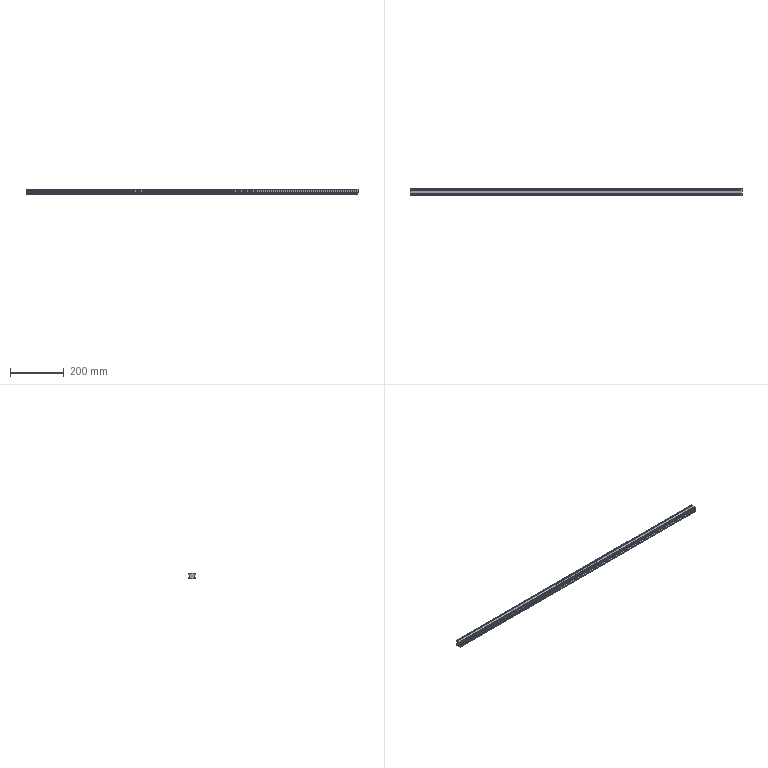Component | SolidWorks | GuideRailHGH25-1 | 1 solid | 34 faces | box 1240 x 23 x 22 mm | volume 545518 mm3 | plane 30 | cylinder 4 | commonest cylinder face diameters 4.6 x4
build123d program:
from build123d import *

# Parameters (mm, degrees)
BOSS_EXTRUDE1_DEPTH = 620


with BuildPart() as part:
    # Sketch1 → Boss-Extrude1 (new, symmetric)
    with BuildSketch(Plane.XY):
        with BuildLine():
            Line((-10.5, 0), (-8.214, 0))
            Line((-8.214, 0), (-7.448, 0.7667))
            Line((-7.448, 0.7667), (-5.695, 0.7667))
            Line((-5.695, 0.7667), (-4.929, 0))
            Line((-4.929, 0), (4.929, 0))
            Line((4.929, 0), (5.695, 0.7667))
            Line((5.695, 0.7667), (7.448, 0.7667))
            Line((7.448, 0.7667), (8.214, 0))
            Line((8.214, 0), (10.5, 0))
            Line((10.5, 0), (11.5, 1))
            Line((11.5, 1), (11.5, 5.5))
            Line((11.5, 5.5), (8.05, 8.95))
            Line((8.05, 8.95), (8.05, 11.95))
            Line((8.05, 11.95), (8.699, 12.599))
            ThreePointArc((8.699, 12.599), (9.368, 14.082), (10.851, 14.751))
            Line((10.851, 14.751), (11.5, 15.4))
            Line((11.5, 15.4), (11.5, 18.55))
            Line((11.5, 18.55), (10.851, 19.199))
            ThreePointArc((10.851, 19.199), (9.368, 19.868), (8.699, 21.351))
            Line((8.699, 21.351), (8.05, 22))
            Line((8.05, 22), (-8.05, 22))
            Line((-8.05, 22), (-8.699, 21.351))
            ThreePointArc((-8.699, 21.351), (-9.368, 19.868), (-10.851, 19.199))
            Line((-10.851, 19.199), (-11.5, 18.55))
            Line((-11.5, 18.55), (-11.5, 15.4))
            Line((-11.5, 15.4), (-10.851, 14.751))
            ThreePointArc((-10.851, 14.751), (-9.368, 14.082), (-8.699, 12.599))
            Line((-8.699, 12.599), (-8.05, 11.95))
            Line((-8.05, 11.95), (-8.05, 8.95))
            Line((-8.05, 8.95), (-11.5, 5.5))
            Line((-11.5, 5.5), (-11.5, 1))
            Line((-11.5, 1), (-10.5, 0))
        make_face()
    extrude(amount=BOSS_EXTRUDE1_DEPTH, both=True)


solid = part.part

# Placed as in the assembly
solid = solid.moved(Location((160, -213.5, 69), (-90, 90, 0)))
STEP:
#1=CARTESIAN_POINT('',(-18.11,-8.748,1.876));
#2=VERTEX_POINT('',#1);
#3=CARTESIAN_POINT('',(-18.11,-8.722,1.85));
#4=VERTEX_POINT('',#3);
#5=CARTESIAN_POINT('',(-18.11,-8.748,1.876));
#6=DIRECTION('',(-0.,0.7071,-0.7071));
#7=VECTOR('',#6,39.37);
#8=LINE('',#5,#7);
#9=EDGE_CURVE('',#2,#4,#8,.T.);
#10=ORIENTED_EDGE('',*,*,#9,.T.);
#11=CARTESIAN_POINT('',(30.709,-8.722,1.85));
#12=VERTEX_POINT('',#11);
#13=CARTESIAN_POINT('',(30.709,-8.722,1.85));
#14=DIRECTION('',(-1.,0.,0.));
#15=VECTOR('',#14,39.37);
#16=LINE('',#13,#15);
#17=EDGE_CURVE('',#12,#4,#16,.T.);
#18=ORIENTED_EDGE('',*,*,#17,.F.);
#19=CARTESIAN_POINT('',(30.709,-8.748,1.876));
#20=VERTEX_POINT('',#19);
#21=CARTESIAN_POINT('',(30.709,-8.748,1.876));
#22=DIRECTION('',(-0.,0.7071,-0.7071));
#23=VECTOR('',#22,39.37);
#24=LINE('',#21,#23);
#25=EDGE_CURVE('',#20,#12,#24,.T.);
#26=ORIENTED_EDGE('',*,*,#25,.F.);
#27=CARTESIAN_POINT('',(30.709,-8.748,1.876));
#28=DIRECTION('',(-1.,0.,0.));
#29=VECTOR('',#28,39.37);
#30=LINE('',#27,#29);
#31=EDGE_CURVE('',#20,#2,#30,.T.);
#32=ORIENTED_EDGE('',*,*,#31,.T.);
#33=EDGE_LOOP('',(#10,#18,#26,#32));
#34=FACE_OUTER_BOUND('',#33,.T.);
#35=CARTESIAN_POINT('',(30.709,-8.748,1.876));
#36=DIRECTION('',(0.,0.7071,0.7071));
#37=DIRECTION('',(0.,-0.7071,0.7071));
#38=AXIS2_PLACEMENT_3D('',#35,#36,#37);
#39=PLANE('',#38);
#40=ADVANCED_FACE('',(#34),#39,.F.);
#41=CARTESIAN_POINT('',(-18.11,-8.089,1.85));
#42=VERTEX_POINT('',#41);
#43=CARTESIAN_POINT('',(-18.11,-8.722,1.85));
#44=DIRECTION('',(0.,1.,0.));
#45=VECTOR('',#44,39.37);
#46=LINE('',#43,#45);
#47=EDGE_CURVE('',#4,#42,#46,.T.);
#48=ORIENTED_EDGE('',*,*,#47,.T.);
#49=CARTESIAN_POINT('',(30.709,-8.089,1.85));
#50=VERTEX_POINT('',#49);
#51=CARTESIAN_POINT('',(30.709,-8.089,1.85));
#52=DIRECTION('',(-1.,0.,0.));
#53=VECTOR('',#52,39.37);
#54=LINE('',#51,#53);
#55=EDGE_CURVE('',#50,#42,#54,.T.);
#56=ORIENTED_EDGE('',*,*,#55,.F.);
#57=CARTESIAN_POINT('',(30.709,-8.722,1.85));
#58=DIRECTION('',(0.,1.,0.));
#59=VECTOR('',#58,39.37);
#60=LINE('',#57,#59);
#61=EDGE_CURVE('',#12,#50,#60,.T.);
#62=ORIENTED_EDGE('',*,*,#61,.F.);
#63=ORIENTED_EDGE('',*,*,#17,.T.);
#64=EDGE_LOOP('',(#48,#56,#62,#63));
#65=FACE_OUTER_BOUND('',#64,.T.);
#66=CARTESIAN_POINT('',(30.709,-8.722,1.85));
#67=DIRECTION('',(0.,-0.,1.));
#68=DIRECTION('',(-0.,-1.,-0.));
#69=AXIS2_PLACEMENT_3D('',#66,#67,#68);
#70=PLANE('',#69);
#71=ADVANCED_FACE('',(#65),#70,.F.);
#72=CARTESIAN_POINT('',(-18.11,-8.063,1.876));
#73=VERTEX_POINT('',#72);
#74=CARTESIAN_POINT('',(-18.11,-8.089,1.85));
#75=DIRECTION('',(0.,0.7071,0.7071));
#76=VECTOR('',#75,39.37);
#77=LINE('',#74,#76);
#78=EDGE_CURVE('',#42,#73,#77,.T.);
#79=ORIENTED_EDGE('',*,*,#78,.T.);
#80=CARTESIAN_POINT('',(30.709,-8.063,1.876));
#81=VERTEX_POINT('',#80);
#82=CARTESIAN_POINT('',(30.709,-8.063,1.876));
#83=DIRECTION('',(-1.,0.,0.));
#84=VECTOR('',#83,39.37);
#85=LINE('',#82,#84);
#86=EDGE_CURVE('',#81,#73,#85,.T.);
#87=ORIENTED_EDGE('',*,*,#86,.F.);
#88=CARTESIAN_POINT('',(30.709,-8.089,1.85));
#89=DIRECTION('',(0.,0.7071,0.7071));
#90=VECTOR('',#89,39.37);
#91=LINE('',#88,#90);
#92=EDGE_CURVE('',#50,#81,#91,.T.);
#93=ORIENTED_EDGE('',*,*,#92,.F.);
#94=ORIENTED_EDGE('',*,*,#55,.T.);
#95=EDGE_LOOP('',(#79,#87,#93,#94));
#96=FACE_OUTER_BOUND('',#95,.T.);
#97=CARTESIAN_POINT('',(30.709,-8.089,1.85));
#98=DIRECTION('',(0.,-0.7071,0.7071));
#99=DIRECTION('',(-0.,-0.7071,-0.7071));
#100=AXIS2_PLACEMENT_3D('',#97,#98,#99);
#101=PLANE('',#100);
#102=ADVANCED_FACE('',(#96),#101,.F.);
#103=CARTESIAN_POINT('',(-18.11,-7.978,1.961));
#104=VERTEX_POINT('',#103);
#105=CARTESIAN_POINT('',(-18.11,-7.973,1.87));
#106=DIRECTION('',(1.,-0.,-0.));
#107=DIRECTION('',(0.,-1.,-0.));
#108=AXIS2_PLACEMENT_3D('',#105,#106,#107);
#109=CIRCLE('',#108,0.09055);
#110=EDGE_CURVE('',#104,#73,#109,.T.);
#111=ORIENTED_EDGE('',*,*,#110,.F.);
#112=CARTESIAN_POINT('',(30.709,-7.978,1.961));
#113=VERTEX_POINT('',#112);
#114=CARTESIAN_POINT('',(30.709,-7.978,1.961));
#115=DIRECTION('',(-1.,0.,0.));
#116=VECTOR('',#115,39.37);
#117=LINE('',#114,#116);
#118=EDGE_CURVE('',#113,#104,#117,.T.);
#119=ORIENTED_EDGE('',*,*,#118,.F.);
#120=CARTESIAN_POINT('',(30.709,-7.973,1.87));
#121=DIRECTION('',(1.,-0.,-0.));
#122=DIRECTION('',(0.,-1.,-0.));
#123=AXIS2_PLACEMENT_3D('',#120,#121,#122);
#124=CIRCLE('',#123,0.09055);
#125=EDGE_CURVE('',#113,#81,#124,.T.);
#126=ORIENTED_EDGE('',*,*,#125,.T.);
#127=ORIENTED_EDGE('',*,*,#86,.T.);
#128=EDGE_LOOP('',(#111,#119,#126,#127));
#129=FACE_OUTER_BOUND('',#128,.T.);
#130=CARTESIAN_POINT('',(30.709,-7.973,1.87));
#131=DIRECTION('',(-1.,0.,0.));
#132=DIRECTION('',(0.,1.,0.));
#133=AXIS2_PLACEMENT_3D('',#130,#131,#132);
#134=CYLINDRICAL_SURFACE('',#133,0.09055);
#135=ADVANCED_FACE('',(#129),#134,.F.);
#136=CARTESIAN_POINT('',(-18.11,-7.953,1.986));
#137=VERTEX_POINT('',#136);
#138=CARTESIAN_POINT('',(-18.11,-7.978,1.961));
#139=DIRECTION('',(0.,0.7071,0.7071));
#140=VECTOR('',#139,39.37);
#141=LINE('',#138,#140);
#142=EDGE_CURVE('',#104,#137,#141,.T.);
#143=ORIENTED_EDGE('',*,*,#142,.T.);
#144=CARTESIAN_POINT('',(30.709,-7.953,1.986));
#145=VERTEX_POINT('',#144);
#146=CARTESIAN_POINT('',(30.709,-7.953,1.986));
#147=DIRECTION('',(-1.,0.,0.));
#148=VECTOR('',#147,39.37);
#149=LINE('',#146,#148);
#150=EDGE_CURVE('',#145,#137,#149,.T.);
#151=ORIENTED_EDGE('',*,*,#150,.F.);
#152=CARTESIAN_POINT('',(30.709,-7.978,1.961));
#153=DIRECTION('',(0.,0.7071,0.7071));
#154=VECTOR('',#153,39.37);
#155=LINE('',#152,#154);
#156=EDGE_CURVE('',#113,#145,#155,.T.);
#157=ORIENTED_EDGE('',*,*,#156,.F.);
#158=ORIENTED_EDGE('',*,*,#118,.T.);
#159=EDGE_LOOP('',(#143,#151,#157,#158));
#160=FACE_OUTER_BOUND('',#159,.T.);
#161=CARTESIAN_POINT('',(30.709,-7.978,1.961));
#162=DIRECTION('',(0.,-0.7071,0.7071));
#163=DIRECTION('',(-0.,-0.7071,-0.7071));
#164=AXIS2_PLACEMENT_3D('',#161,#162,#163);
#165=PLANE('',#164);
#166=ADVANCED_FACE('',(#160),#165,.F.);
#167=CARTESIAN_POINT('',(-18.11,-7.953,2.11));
#168=VERTEX_POINT('',#167);
#169=CARTESIAN_POINT('',(-18.11,-7.953,1.986));
#170=DIRECTION('',(0.,-0.,1.));
#171=VECTOR('',#170,39.37);
#172=LINE('',#169,#171);
#173=EDGE_CURVE('',#137,#168,#172,.T.);
#174=ORIENTED_EDGE('',*,*,#173,.T.);
#175=CARTESIAN_POINT('',(30.709,-7.953,2.11));
#176=VERTEX_POINT('',#175);
#177=CARTESIAN_POINT('',(30.709,-7.953,2.11));
#178=DIRECTION('',(-1.,0.,0.));
#179=VECTOR('',#178,39.37);
#180=LINE('',#177,#179);
#181=EDGE_CURVE('',#176,#168,#180,.T.);
#182=ORIENTED_EDGE('',*,*,#181,.F.);
#183=CARTESIAN_POINT('',(30.709,-7.953,1.986));
#184=DIRECTION('',(0.,-0.,1.));
#185=VECTOR('',#184,39.37);
#186=LINE('',#183,#185);
#187=EDGE_CURVE('',#145,#176,#186,.T.);
#188=ORIENTED_EDGE('',*,*,#187,.F.);
#189=ORIENTED_EDGE('',*,*,#150,.T.);
#190=EDGE_LOOP('',(#174,#182,#188,#189));
#191=FACE_OUTER_BOUND('',#190,.T.);
#192=CARTESIAN_POINT('',(30.709,-7.953,1.986));
#193=DIRECTION('',(-0.,-1.,-0.));
#194=DIRECTION('',(-1.,0.,0.));
#195=AXIS2_PLACEMENT_3D('',#192,#193,#194);
#196=PLANE('',#195);
#197=ADVANCED_FACE('',(#191),#196,.F.);
#198=CARTESIAN_POINT('',(-18.11,-7.978,2.136));
#199=VERTEX_POINT('',#198);
#200=CARTESIAN_POINT('',(-18.11,-7.953,2.11));
#201=DIRECTION('',(0.,-0.7071,0.7071));
#202=VECTOR('',#201,39.37);
#203=LINE('',#200,#202);
#204=EDGE_CURVE('',#168,#199,#203,.T.);
#205=ORIENTED_EDGE('',*,*,#204,.T.);
#206=CARTESIAN_POINT('',(30.709,-7.978,2.136));
#207=VERTEX_POINT('',#206);
#208=CARTESIAN_POINT('',(30.709,-7.978,2.136));
#209=DIRECTION('',(-1.,0.,0.));
#210=VECTOR('',#209,39.37);
#211=LINE('',#208,#210);
#212=EDGE_CURVE('',#207,#199,#211,.T.);
#213=ORIENTED_EDGE('',*,*,#212,.F.);
#214=CARTESIAN_POINT('',(30.709,-7.953,2.11));
#215=DIRECTION('',(0.,-0.7071,0.7071));
#216=VECTOR('',#215,39.37);
#217=LINE('',#214,#216);
#218=EDGE_CURVE('',#176,#207,#217,.T.);
#219=ORIENTED_EDGE('',*,*,#218,.F.);
#220=ORIENTED_EDGE('',*,*,#181,.T.);
#221=EDGE_LOOP('',(#205,#213,#219,#220));
#222=FACE_OUTER_BOUND('',#221,.T.);
#223=CARTESIAN_POINT('',(30.709,-7.953,2.11));
#224=DIRECTION('',(-0.,-0.7071,-0.7071));
#225=DIRECTION('',(-0.,0.7071,-0.7071));
#226=AXIS2_PLACEMENT_3D('',#223,#224,#225);
#227=PLANE('',#226);
#228=ADVANCED_FACE('',(#222),#227,.F.);
#229=CARTESIAN_POINT('',(-18.11,-8.063,2.221));
#230=VERTEX_POINT('',#229);
#231=CARTESIAN_POINT('',(-18.11,-7.973,2.226));
#232=DIRECTION('',(1.,-0.,-0.));
#233=DIRECTION('',(0.,-1.,-0.));
#234=AXIS2_PLACEMENT_3D('',#231,#232,#233);
#235=CIRCLE('',#234,0.09055);
#236=EDGE_CURVE('',#230,#199,#235,.T.);
#237=ORIENTED_EDGE('',*,*,#236,.F.);
#238=CARTESIAN_POINT('',(30.709,-8.063,2.221));
#239=VERTEX_POINT('',#238);
#240=CARTESIAN_POINT('',(30.709,-8.063,2.221));
#241=DIRECTION('',(-1.,0.,0.));
#242=VECTOR('',#241,39.37);
#243=LINE('',#240,#242);
#244=EDGE_CURVE('',#239,#230,#243,.T.);
#245=ORIENTED_EDGE('',*,*,#244,.F.);
#246=CARTESIAN_POINT('',(30.709,-7.973,2.226));
#247=DIRECTION('',(1.,-0.,-0.));
#248=DIRECTION('',(0.,-1.,-0.));
#249=AXIS2_PLACEMENT_3D('',#246,#247,#248);
#250=CIRCLE('',#249,0.09055);
#251=EDGE_CURVE('',#239,#207,#250,.T.);
#252=ORIENTED_EDGE('',*,*,#251,.T.);
#253=ORIENTED_EDGE('',*,*,#212,.T.);
#254=EDGE_LOOP('',(#237,#245,#252,#253));
#255=FACE_OUTER_BOUND('',#254,.T.);
#256=CARTESIAN_POINT('',(30.709,-7.973,2.226));
#257=DIRECTION('',(-1.,0.,0.));
#258=DIRECTION('',(0.,1.,0.));
#259=AXIS2_PLACEMENT_3D('',#256,#257,#258);
#260=CYLINDRICAL_SURFACE('',#259,0.09055);
#261=ADVANCED_FACE('',(#255),#260,.F.);
#262=CARTESIAN_POINT('',(-18.11,-8.089,2.246));
#263=VERTEX_POINT('',#262);
#264=CARTESIAN_POINT('',(-18.11,-8.063,2.221));
#265=DIRECTION('',(0.,-0.7071,0.7071));
#266=VECTOR('',#265,39.37);
#267=LINE('',#264,#266);
#268=EDGE_CURVE('',#230,#263,#267,.T.);
#269=ORIENTED_EDGE('',*,*,#268,.T.);
#270=CARTESIAN_POINT('',(30.709,-8.089,2.246));
#271=VERTEX_POINT('',#270);
#272=CARTESIAN_POINT('',(30.709,-8.089,2.246));
#273=DIRECTION('',(-1.,0.,0.));
#274=VECTOR('',#273,39.37);
#275=LINE('',#272,#274);
#276=EDGE_CURVE('',#271,#263,#275,.T.);
#277=ORIENTED_EDGE('',*,*,#276,.F.);
#278=CARTESIAN_POINT('',(30.709,-8.063,2.221));
#279=DIRECTION('',(0.,-0.7071,0.7071));
#280=VECTOR('',#279,39.37);
#281=LINE('',#278,#280);
#282=EDGE_CURVE('',#239,#271,#281,.T.);
#283=ORIENTED_EDGE('',*,*,#282,.F.);
#284=ORIENTED_EDGE('',*,*,#244,.T.);
#285=EDGE_LOOP('',(#269,#277,#283,#284));
#286=FACE_OUTER_BOUND('',#285,.T.);
#287=CARTESIAN_POINT('',(30.709,-8.063,2.221));
#288=DIRECTION('',(-0.,-0.7071,-0.7071));
#289=DIRECTION('',(-0.,0.7071,-0.7071));
#290=AXIS2_PLACEMENT_3D('',#287,#288,#289);
#291=PLANE('',#290);
#292=ADVANCED_FACE('',(#286),#291,.F.);
#293=CARTESIAN_POINT('',(-18.11,-8.089,2.364));
#294=VERTEX_POINT('',#293);
#295=CARTESIAN_POINT('',(-18.11,-8.089,2.246));
#296=DIRECTION('',(0.,-0.,1.));
#297=VECTOR('',#296,39.37);
#298=LINE('',#295,#297);
#299=EDGE_CURVE('',#263,#294,#298,.T.);
#300=ORIENTED_EDGE('',*,*,#299,.T.);
#301=CARTESIAN_POINT('',(30.709,-8.089,2.364));
#302=VERTEX_POINT('',#301);
#303=CARTESIAN_POINT('',(30.709,-8.089,2.364));
#304=DIRECTION('',(-1.,0.,0.));
#305=VECTOR('',#304,39.37);
#306=LINE('',#303,#305);
#307=EDGE_CURVE('',#302,#294,#306,.T.);
#308=ORIENTED_EDGE('',*,*,#307,.F.);
#309=CARTESIAN_POINT('',(30.709,-8.089,2.246));
#310=DIRECTION('',(0.,-0.,1.));
#311=VECTOR('',#310,39.37);
#312=LINE('',#309,#311);
#313=EDGE_CURVE('',#271,#302,#312,.T.);
#314=ORIENTED_EDGE('',*,*,#313,.F.);
#315=ORIENTED_EDGE('',*,*,#276,.T.);
#316=EDGE_LOOP('',(#300,#308,#314,#315));
#317=FACE_OUTER_BOUND('',#316,.T.);
#318=CARTESIAN_POINT('',(30.709,-8.089,2.246));
#319=DIRECTION('',(-0.,-1.,-0.));
#320=DIRECTION('',(-0.,0.,-1.));
#321=AXIS2_PLACEMENT_3D('',#318,#319,#320);
#322=PLANE('',#321);
#323=ADVANCED_FACE('',(#317),#322,.F.);
#324=CARTESIAN_POINT('',(-18.11,-7.953,2.5));
#325=VERTEX_POINT('',#324);
#326=CARTESIAN_POINT('',(-18.11,-8.089,2.364));
#327=DIRECTION('',(0.,0.7071,0.7071));
#328=VECTOR('',#327,39.37);
#329=LINE('',#326,#328);
#330=EDGE_CURVE('',#294,#325,#329,.T.);
#331=ORIENTED_EDGE('',*,*,#330,.T.);
#332=CARTESIAN_POINT('',(30.709,-7.953,2.5));
#333=VERTEX_POINT('',#332);
#334=CARTESIAN_POINT('',(30.709,-7.953,2.5));
#335=DIRECTION('',(-1.,0.,0.));
#336=VECTOR('',#335,39.37);
#337=LINE('',#334,#336);
#338=EDGE_CURVE('',#333,#325,#337,.T.);
#339=ORIENTED_EDGE('',*,*,#338,.F.);
#340=CARTESIAN_POINT('',(30.709,-8.089,2.364));
#341=DIRECTION('',(0.,0.7071,0.7071));
#342=VECTOR('',#341,39.37);
#343=LINE('',#340,#342);
#344=EDGE_CURVE('',#302,#333,#343,.T.);
#345=ORIENTED_EDGE('',*,*,#344,.F.);
#346=ORIENTED_EDGE('',*,*,#307,.T.);
#347=EDGE_LOOP('',(#331,#339,#345,#346));
#348=FACE_OUTER_BOUND('',#347,.T.);
#349=CARTESIAN_POINT('',(30.709,-8.089,2.364));
#350=DIRECTION('',(0.,-0.7071,0.7071));
#351=DIRECTION('',(-0.,-0.7071,-0.7071));
#352=AXIS2_PLACEMENT_3D('',#349,#350,#351);
#353=PLANE('',#352);
#354=ADVANCED_FACE('',(#348),#353,.F.);
#355=CARTESIAN_POINT('',(-18.11,-7.953,2.677));
#356=VERTEX_POINT('',#355);
#357=CARTESIAN_POINT('',(-18.11,-7.953,2.5));
#358=DIRECTION('',(0.,-0.,1.));
#359=VECTOR('',#358,39.37);
#360=LINE('',#357,#359);
#361=EDGE_CURVE('',#325,#356,#360,.T.);
#362=ORIENTED_EDGE('',*,*,#361,.T.);
#363=CARTESIAN_POINT('',(30.709,-7.953,2.677));
#364=VERTEX_POINT('',#363);
#365=CARTESIAN_POINT('',(30.709,-7.953,2.677));
#366=DIRECTION('',(-1.,0.,0.));
#367=VECTOR('',#366,39.37);
#368=LINE('',#365,#367);
#369=EDGE_CURVE('',#364,#356,#368,.T.);
#370=ORIENTED_EDGE('',*,*,#369,.F.);
#371=CARTESIAN_POINT('',(30.709,-7.953,2.5));
#372=DIRECTION('',(0.,-0.,1.));
#373=VECTOR('',#372,39.37);
#374=LINE('',#371,#373);
#375=EDGE_CURVE('',#333,#364,#374,.T.);
#376=ORIENTED_EDGE('',*,*,#375,.F.);
#377=ORIENTED_EDGE('',*,*,#338,.T.);
#378=EDGE_LOOP('',(#362,#370,#376,#377));
#379=FACE_OUTER_BOUND('',#378,.T.);
#380=CARTESIAN_POINT('',(30.709,-7.953,2.5));
#381=DIRECTION('',(-0.,-1.,-0.));
#382=DIRECTION('',(-1.,0.,0.));
#383=AXIS2_PLACEMENT_3D('',#380,#381,#382);
#384=PLANE('',#383);
#385=ADVANCED_FACE('',(#379),#384,.F.);
#386=CARTESIAN_POINT('',(-18.11,-7.992,2.717));
#387=VERTEX_POINT('',#386);
#388=CARTESIAN_POINT('',(-18.11,-7.953,2.677));
#389=DIRECTION('',(0.,-0.7071,0.7071));
#390=VECTOR('',#389,39.37);
#391=LINE('',#388,#390);
#392=EDGE_CURVE('',#356,#387,#391,.T.);
#393=ORIENTED_EDGE('',*,*,#392,.T.);
#394=CARTESIAN_POINT('',(30.709,-7.992,2.717));
#395=VERTEX_POINT('',#394);
#396=CARTESIAN_POINT('',(30.709,-7.992,2.717));
#397=DIRECTION('',(-1.,0.,0.));
#398=VECTOR('',#397,39.37);
#399=LINE('',#396,#398);
#400=EDGE_CURVE('',#395,#387,#399,.T.);
#401=ORIENTED_EDGE('',*,*,#400,.F.);
#402=CARTESIAN_POINT('',(30.709,-7.953,2.677));
#403=DIRECTION('',(0.,-0.7071,0.7071));
#404=VECTOR('',#403,39.37);
#405=LINE('',#402,#404);
#406=EDGE_CURVE('',#364,#395,#405,.T.);
#407=ORIENTED_EDGE('',*,*,#406,.F.);
#408=ORIENTED_EDGE('',*,*,#369,.T.);
#409=EDGE_LOOP('',(#393,#401,#407,#408));
#410=FACE_OUTER_BOUND('',#409,.T.);
#411=CARTESIAN_POINT('',(30.709,-7.953,2.677));
#412=DIRECTION('',(-0.,-0.7071,-0.7071));
#413=DIRECTION('',(-0.,0.7071,-0.7071));
#414=AXIS2_PLACEMENT_3D('',#411,#412,#413);
#415=PLANE('',#414);
#416=ADVANCED_FACE('',(#410),#415,.F.);
#417=CARTESIAN_POINT('',(-18.11,-8.082,2.717));
#418=VERTEX_POINT('',#417);
#419=CARTESIAN_POINT('',(-18.11,-7.992,2.717));
#420=DIRECTION('',(-0.,-1.,0.));
#421=VECTOR('',#420,39.37);
#422=LINE('',#419,#421);
#423=EDGE_CURVE('',#387,#418,#422,.T.);
#424=ORIENTED_EDGE('',*,*,#423,.T.);
#425=CARTESIAN_POINT('',(30.709,-8.082,2.717));
#426=VERTEX_POINT('',#425);
#427=CARTESIAN_POINT('',(30.709,-8.082,2.717));
#428=DIRECTION('',(-1.,0.,0.));
#429=VECTOR('',#428,39.37);
#430=LINE('',#427,#429);
#431=EDGE_CURVE('',#426,#418,#430,.T.);
#432=ORIENTED_EDGE('',*,*,#431,.F.);
#433=CARTESIAN_POINT('',(30.709,-7.992,2.717));
#434=DIRECTION('',(-0.,-1.,0.));
#435=VECTOR('',#434,39.37);
#436=LINE('',#433,#435);
#437=EDGE_CURVE('',#395,#426,#436,.T.);
#438=ORIENTED_EDGE('',*,*,#437,.F.);
#439=ORIENTED_EDGE('',*,*,#400,.T.);
#440=EDGE_LOOP('',(#424,#432,#438,#439));
#441=FACE_OUTER_BOUND('',#440,.T.);
#442=CARTESIAN_POINT('',(30.709,-7.992,2.717));
#443=DIRECTION('',(-0.,-0.,-1.));
#444=DIRECTION('',(0.,1.,-0.));
#445=AXIS2_PLACEMENT_3D('',#442,#443,#444);
#446=PLANE('',#445);
#447=ADVANCED_FACE('',(#441),#446,.F.);
#448=CARTESIAN_POINT('',(-18.11,-8.112,2.686));
#449=VERTEX_POINT('',#448);
#450=CARTESIAN_POINT('',(-18.11,-8.082,2.717));
#451=DIRECTION('',(-0.,-0.7071,-0.7071));
#452=VECTOR('',#451,39.37);
#453=LINE('',#450,#452);
#454=EDGE_CURVE('',#418,#449,#453,.T.);
#455=ORIENTED_EDGE('',*,*,#454,.T.);
#456=CARTESIAN_POINT('',(30.709,-8.112,2.686));
#457=VERTEX_POINT('',#456);
#458=CARTESIAN_POINT('',(30.709,-8.112,2.686));
#459=DIRECTION('',(-1.,0.,0.));
#460=VECTOR('',#459,39.37);
#461=LINE('',#458,#460);
#462=EDGE_CURVE('',#457,#449,#461,.T.);
#463=ORIENTED_EDGE('',*,*,#462,.F.);
#464=CARTESIAN_POINT('',(30.709,-8.082,2.717));
#465=DIRECTION('',(-0.,-0.7071,-0.7071));
#466=VECTOR('',#465,39.37);
#467=LINE('',#464,#466);
#468=EDGE_CURVE('',#426,#457,#467,.T.);
#469=ORIENTED_EDGE('',*,*,#468,.F.);
#470=ORIENTED_EDGE('',*,*,#431,.T.);
#471=EDGE_LOOP('',(#455,#463,#469,#470));
#472=FACE_OUTER_BOUND('',#471,.T.);
#473=CARTESIAN_POINT('',(30.709,-8.082,2.717));
#474=DIRECTION('',(-0.,0.7071,-0.7071));
#475=DIRECTION('',(0.,0.7071,0.7071));
#476=AXIS2_PLACEMENT_3D('',#473,#474,#475);
#477=PLANE('',#476);
#478=ADVANCED_FACE('',(#472),#477,.F.);
#479=CARTESIAN_POINT('',(-18.11,-8.181,2.686));
#480=VERTEX_POINT('',#479);
#481=CARTESIAN_POINT('',(-18.11,-8.112,2.686));
#482=DIRECTION('',(-0.,-1.,-0.));
#483=VECTOR('',#482,39.37);
#484=LINE('',#481,#483);
#485=EDGE_CURVE('',#449,#480,#484,.T.);
#486=ORIENTED_EDGE('',*,*,#485,.T.);
#487=CARTESIAN_POINT('',(30.709,-8.181,2.686));
#488=VERTEX_POINT('',#487);
#489=CARTESIAN_POINT('',(30.709,-8.181,2.686));
#490=DIRECTION('',(-1.,0.,0.));
#491=VECTOR('',#490,39.37);
#492=LINE('',#489,#491);
#493=EDGE_CURVE('',#488,#480,#492,.T.);
#494=ORIENTED_EDGE('',*,*,#493,.F.);
#495=CARTESIAN_POINT('',(30.709,-8.112,2.686));
#496=DIRECTION('',(-0.,-1.,-0.));
#497=VECTOR('',#496,39.37);
#498=LINE('',#495,#497);
#499=EDGE_CURVE('',#457,#488,#498,.T.);
#500=ORIENTED_EDGE('',*,*,#499,.F.);
#501=ORIENTED_EDGE('',*,*,#462,.T.);
#502=EDGE_LOOP('',(#486,#494,#500,#501));
#503=FACE_OUTER_BOUND('',#502,.T.);
#504=CARTESIAN_POINT('',(30.709,-8.112,2.686));
#505=DIRECTION('',(-0.,0.,-1.));
#506=DIRECTION('',(0.,1.,0.));
#507=AXIS2_PLACEMENT_3D('',#504,#505,#506);
#508=PLANE('',#507);
#509=ADVANCED_FACE('',(#503),#508,.F.);
#510=CARTESIAN_POINT('',(-18.11,-8.211,2.717));
#511=VERTEX_POINT('',#510);
#512=CARTESIAN_POINT('',(-18.11,-8.181,2.686));
#513=DIRECTION('',(0.,-0.7071,0.7071));
#514=VECTOR('',#513,39.37);
#515=LINE('',#512,#514);
#516=EDGE_CURVE('',#480,#511,#515,.T.);
#517=ORIENTED_EDGE('',*,*,#516,.T.);
#518=CARTESIAN_POINT('',(30.709,-8.211,2.717));
#519=VERTEX_POINT('',#518);
#520=CARTESIAN_POINT('',(30.709,-8.211,2.717));
#521=DIRECTION('',(-1.,0.,0.));
#522=VECTOR('',#521,39.37);
#523=LINE('',#520,#522);
#524=EDGE_CURVE('',#519,#511,#523,.T.);
#525=ORIENTED_EDGE('',*,*,#524,.F.);
#526=CARTESIAN_POINT('',(30.709,-8.181,2.686));
#527=DIRECTION('',(0.,-0.7071,0.7071));
#528=VECTOR('',#527,39.37);
#529=LINE('',#526,#528);
#530=EDGE_CURVE('',#488,#519,#529,.T.);
#531=ORIENTED_EDGE('',*,*,#530,.F.);
#532=ORIENTED_EDGE('',*,*,#493,.T.);
#533=EDGE_LOOP('',(#517,#525,#531,#532));
#534=FACE_OUTER_BOUND('',#533,.T.);
#535=CARTESIAN_POINT('',(30.709,-8.181,2.686));
#536=DIRECTION('',(-0.,-0.7071,-0.7071));
#537=DIRECTION('',(-0.,0.7071,-0.7071));
#538=AXIS2_PLACEMENT_3D('',#535,#536,#537);
#539=PLANE('',#538);
#540=ADVANCED_FACE('',(#534),#539,.F.);
#541=CARTESIAN_POINT('',(-18.11,-8.6,2.717));
#542=VERTEX_POINT('',#541);
#543=CARTESIAN_POINT('',(-18.11,-8.211,2.717));
#544=DIRECTION('',(-0.,-1.,-0.));
#545=VECTOR('',#544,39.37);
#546=LINE('',#543,#545);
#547=EDGE_CURVE('',#511,#542,#546,.T.);
#548=ORIENTED_EDGE('',*,*,#547,.T.);
#549=CARTESIAN_POINT('',(30.709,-8.6,2.717));
#550=VERTEX_POINT('',#549);
#551=CARTESIAN_POINT('',(30.709,-8.6,2.717));
#552=DIRECTION('',(-1.,0.,0.));
#553=VECTOR('',#552,39.37);
#554=LINE('',#551,#553);
#555=EDGE_CURVE('',#550,#542,#554,.T.);
#556=ORIENTED_EDGE('',*,*,#555,.F.);
#557=CARTESIAN_POINT('',(30.709,-8.211,2.717));
#558=DIRECTION('',(-0.,-1.,-0.));
#559=VECTOR('',#558,39.37);
#560=LINE('',#557,#559);
#561=EDGE_CURVE('',#519,#550,#560,.T.);
#562=ORIENTED_EDGE('',*,*,#561,.F.);
#563=ORIENTED_EDGE('',*,*,#524,.T.);
#564=EDGE_LOOP('',(#548,#556,#562,#563));
#565=FACE_OUTER_BOUND('',#564,.T.);
#566=CARTESIAN_POINT('',(30.709,-8.211,2.717));
#567=DIRECTION('',(-0.,0.,-1.));
#568=DIRECTION('',(0.,1.,0.));
#569=AXIS2_PLACEMENT_3D('',#566,#567,#568);
#570=PLANE('',#569);
#571=ADVANCED_FACE('',(#565),#570,.F.);
#572=CARTESIAN_POINT('',(-18.11,-8.63,2.686));
#573=VERTEX_POINT('',#572);
#574=CARTESIAN_POINT('',(-18.11,-8.6,2.717));
#575=DIRECTION('',(-0.,-0.7071,-0.7071));
#576=VECTOR('',#575,39.37);
#577=LINE('',#574,#576);
#578=EDGE_CURVE('',#542,#573,#577,.T.);
#579=ORIENTED_EDGE('',*,*,#578,.T.);
#580=CARTESIAN_POINT('',(30.709,-8.63,2.686));
#581=VERTEX_POINT('',#580);
#582=CARTESIAN_POINT('',(30.709,-8.63,2.686));
#583=DIRECTION('',(-1.,0.,0.));
#584=VECTOR('',#583,39.37);
#585=LINE('',#582,#584);
#586=EDGE_CURVE('',#581,#573,#585,.T.);
#587=ORIENTED_EDGE('',*,*,#586,.F.);
#588=CARTESIAN_POINT('',(30.709,-8.6,2.717));
#589=DIRECTION('',(-0.,-0.7071,-0.7071));
#590=VECTOR('',#589,39.37);
#591=LINE('',#588,#590);
#592=EDGE_CURVE('',#550,#581,#591,.T.);
#593=ORIENTED_EDGE('',*,*,#592,.F.);
#594=ORIENTED_EDGE('',*,*,#555,.T.);
#595=EDGE_LOOP('',(#579,#587,#593,#594));
#596=FACE_OUTER_BOUND('',#595,.T.);
#597=CARTESIAN_POINT('',(30.709,-8.6,2.717));
#598=DIRECTION('',(-0.,0.7071,-0.7071));
#599=DIRECTION('',(0.,0.7071,0.7071));
#600=AXIS2_PLACEMENT_3D('',#597,#598,#599);
#601=PLANE('',#600);
#602=ADVANCED_FACE('',(#596),#601,.F.);
#603=CARTESIAN_POINT('',(-18.11,-8.699,2.686));
#604=VERTEX_POINT('',#603);
#605=CARTESIAN_POINT('',(-18.11,-8.63,2.686));
#606=DIRECTION('',(-0.,-1.,0.));
#607=VECTOR('',#606,39.37);
#608=LINE('',#605,#607);
#609=EDGE_CURVE('',#573,#604,#608,.T.);
#610=ORIENTED_EDGE('',*,*,#609,.T.);
#611=CARTESIAN_POINT('',(30.709,-8.699,2.686));
#612=VERTEX_POINT('',#611);
#613=CARTESIAN_POINT('',(30.709,-8.699,2.686));
#614=DIRECTION('',(-1.,0.,0.));
#615=VECTOR('',#614,39.37);
#616=LINE('',#613,#615);
#617=EDGE_CURVE('',#612,#604,#616,.T.);
#618=ORIENTED_EDGE('',*,*,#617,.F.);
#619=CARTESIAN_POINT('',(30.709,-8.63,2.686));
#620=DIRECTION('',(-0.,-1.,0.));
#621=VECTOR('',#620,39.37);
#622=LINE('',#619,#621);
#623=EDGE_CURVE('',#581,#612,#622,.T.);
#624=ORIENTED_EDGE('',*,*,#623,.F.);
#625=ORIENTED_EDGE('',*,*,#586,.T.);
#626=EDGE_LOOP('',(#610,#618,#624,#625));
#627=FACE_OUTER_BOUND('',#626,.T.);
#628=CARTESIAN_POINT('',(30.709,-8.63,2.686));
#629=DIRECTION('',(-0.,-0.,-1.));
#630=DIRECTION('',(0.,1.,-0.));
#631=AXIS2_PLACEMENT_3D('',#628,#629,#630);
#632=PLANE('',#631);
#633=ADVANCED_FACE('',(#627),#632,.F.);
#634=CARTESIAN_POINT('',(-18.11,-8.729,2.717));
#635=VERTEX_POINT('',#634);
#636=CARTESIAN_POINT('',(-18.11,-8.699,2.686));
#637=DIRECTION('',(0.,-0.7071,0.7071));
#638=VECTOR('',#637,39.37);
#639=LINE('',#636,#638);
#640=EDGE_CURVE('',#604,#635,#639,.T.);
#641=ORIENTED_EDGE('',*,*,#640,.T.);
#642=CARTESIAN_POINT('',(30.709,-8.729,2.717));
#643=VERTEX_POINT('',#642);
#644=CARTESIAN_POINT('',(30.709,-8.729,2.717));
#645=DIRECTION('',(-1.,0.,0.));
#646=VECTOR('',#645,39.37);
#647=LINE('',#644,#646);
#648=EDGE_CURVE('',#643,#635,#647,.T.);
#649=ORIENTED_EDGE('',*,*,#648,.F.);
#650=CARTESIAN_POINT('',(30.709,-8.699,2.686));
#651=DIRECTION('',(0.,-0.7071,0.7071));
#652=VECTOR('',#651,39.37);
#653=LINE('',#650,#652);
#654=EDGE_CURVE('',#612,#643,#653,.T.);
#655=ORIENTED_EDGE('',*,*,#654,.F.);
#656=ORIENTED_EDGE('',*,*,#617,.T.);
#657=EDGE_LOOP('',(#641,#649,#655,#656));
#658=FACE_OUTER_BOUND('',#657,.T.);
#659=CARTESIAN_POINT('',(30.709,-8.699,2.686));
#660=DIRECTION('',(-0.,-0.7071,-0.7071));
#661=DIRECTION('',(-0.,0.7071,-0.7071));
#662=AXIS2_PLACEMENT_3D('',#659,#660,#661);
#663=PLANE('',#662);
#664=ADVANCED_FACE('',(#658),#663,.F.);
#665=CARTESIAN_POINT('',(-18.11,-8.819,2.717));
#666=VERTEX_POINT('',#665);
#667=CARTESIAN_POINT('',(-18.11,-8.729,2.717));
#668=DIRECTION('',(-0.,-1.,-0.));
#669=VECTOR('',#668,39.37);
#670=LINE('',#667,#669);
#671=EDGE_CURVE('',#635,#666,#670,.T.);
#672=ORIENTED_EDGE('',*,*,#671,.T.);
#673=CARTESIAN_POINT('',(30.709,-8.819,2.717));
#674=VERTEX_POINT('',#673);
#675=CARTESIAN_POINT('',(30.709,-8.819,2.717));
#676=DIRECTION('',(-1.,0.,0.));
#677=VECTOR('',#676,39.37);
#678=LINE('',#675,#677);
#679=EDGE_CURVE('',#674,#666,#678,.T.);
#680=ORIENTED_EDGE('',*,*,#679,.F.);
#681=CARTESIAN_POINT('',(30.709,-8.729,2.717));
#682=DIRECTION('',(-0.,-1.,-0.));
#683=VECTOR('',#682,39.37);
#684=LINE('',#681,#683);
#685=EDGE_CURVE('',#643,#674,#684,.T.);
#686=ORIENTED_EDGE('',*,*,#685,.F.);
#687=ORIENTED_EDGE('',*,*,#648,.T.);
#688=EDGE_LOOP('',(#672,#680,#686,#687));
#689=FACE_OUTER_BOUND('',#688,.T.);
#690=CARTESIAN_POINT('',(30.709,-8.729,2.717));
#691=DIRECTION('',(-0.,0.,-1.));
#692=DIRECTION('',(0.,1.,0.));
#693=AXIS2_PLACEMENT_3D('',#690,#691,#692);
#694=PLANE('',#693);
#695=ADVANCED_FACE('',(#689),#694,.F.);
#696=CARTESIAN_POINT('',(-18.11,-8.858,2.677));
#697=VERTEX_POINT('',#696);
#698=CARTESIAN_POINT('',(-18.11,-8.819,2.717));
#699=DIRECTION('',(-0.,-0.7071,-0.7071));
#700=VECTOR('',#699,39.37);
#701=LINE('',#698,#700);
#702=EDGE_CURVE('',#666,#697,#701,.T.);
#703=ORIENTED_EDGE('',*,*,#702,.T.);
#704=CARTESIAN_POINT('',(30.709,-8.858,2.677));
#705=VERTEX_POINT('',#704);
#706=CARTESIAN_POINT('',(30.709,-8.858,2.677));
#707=DIRECTION('',(-1.,0.,0.));
#708=VECTOR('',#707,39.37);
#709=LINE('',#706,#708);
#710=EDGE_CURVE('',#705,#697,#709,.T.);
#711=ORIENTED_EDGE('',*,*,#710,.F.);
#712=CARTESIAN_POINT('',(30.709,-8.819,2.717));
#713=DIRECTION('',(-0.,-0.7071,-0.7071));
#714=VECTOR('',#713,39.37);
#715=LINE('',#712,#714);
#716=EDGE_CURVE('',#674,#705,#715,.T.);
#717=ORIENTED_EDGE('',*,*,#716,.F.);
#718=ORIENTED_EDGE('',*,*,#679,.T.);
#719=EDGE_LOOP('',(#703,#711,#717,#718));
#720=FACE_OUTER_BOUND('',#719,.T.);
#721=CARTESIAN_POINT('',(30.709,-8.819,2.717));
#722=DIRECTION('',(-0.,0.7071,-0.7071));
#723=DIRECTION('',(0.,0.7071,0.7071));
#724=AXIS2_PLACEMENT_3D('',#721,#722,#723);
#725=PLANE('',#724);
#726=ADVANCED_FACE('',(#720),#725,.F.);
#727=CARTESIAN_POINT('',(-18.11,-8.858,2.5));
#728=VERTEX_POINT('',#727);
#729=CARTESIAN_POINT('',(-18.11,-8.858,2.677));
#730=DIRECTION('',(-0.,0.,-1.));
#731=VECTOR('',#730,39.37);
#732=LINE('',#729,#731);
#733=EDGE_CURVE('',#697,#728,#732,.T.);
#734=ORIENTED_EDGE('',*,*,#733,.T.);
#735=CARTESIAN_POINT('',(30.709,-8.858,2.5));
#736=VERTEX_POINT('',#735);
#737=CARTESIAN_POINT('',(30.709,-8.858,2.5));
#738=DIRECTION('',(-1.,0.,0.));
#739=VECTOR('',#738,39.37);
#740=LINE('',#737,#739);
#741=EDGE_CURVE('',#736,#728,#740,.T.);
#742=ORIENTED_EDGE('',*,*,#741,.F.);
#743=CARTESIAN_POINT('',(30.709,-8.858,2.677));
#744=DIRECTION('',(-0.,0.,-1.));
#745=VECTOR('',#744,39.37);
#746=LINE('',#743,#745);
#747=EDGE_CURVE('',#705,#736,#746,.T.);
#748=ORIENTED_EDGE('',*,*,#747,.F.);
#749=ORIENTED_EDGE('',*,*,#710,.T.);
#750=EDGE_LOOP('',(#734,#742,#748,#749));
#751=FACE_OUTER_BOUND('',#750,.T.);
#752=CARTESIAN_POINT('',(30.709,-8.858,2.677));
#753=DIRECTION('',(0.,1.,0.));
#754=DIRECTION('',(0.,-0.,1.));
#755=AXIS2_PLACEMENT_3D('',#752,#753,#754);
#756=PLANE('',#755);
#757=ADVANCED_FACE('',(#751),#756,.F.);
#758=CARTESIAN_POINT('',(-18.11,-8.722,2.364));
#759=VERTEX_POINT('',#758);
#760=CARTESIAN_POINT('',(-18.11,-8.858,2.5));
#761=DIRECTION('',(-0.,0.7071,-0.7071));
#762=VECTOR('',#761,39.37);
#763=LINE('',#760,#762);
#764=EDGE_CURVE('',#728,#759,#763,.T.);
#765=ORIENTED_EDGE('',*,*,#764,.T.);
#766=CARTESIAN_POINT('',(30.709,-8.722,2.364));
#767=VERTEX_POINT('',#766);
#768=CARTESIAN_POINT('',(30.709,-8.722,2.364));
#769=DIRECTION('',(-1.,0.,0.));
#770=VECTOR('',#769,39.37);
#771=LINE('',#768,#770);
#772=EDGE_CURVE('',#767,#759,#771,.T.);
#773=ORIENTED_EDGE('',*,*,#772,.F.);
#774=CARTESIAN_POINT('',(30.709,-8.858,2.5));
#775=DIRECTION('',(-0.,0.7071,-0.7071));
#776=VECTOR('',#775,39.37);
#777=LINE('',#774,#776);
#778=EDGE_CURVE('',#736,#767,#777,.T.);
#779=ORIENTED_EDGE('',*,*,#778,.F.);
#780=ORIENTED_EDGE('',*,*,#741,.T.);
#781=EDGE_LOOP('',(#765,#773,#779,#780));
#782=FACE_OUTER_BOUND('',#781,.T.);
#783=CARTESIAN_POINT('',(30.709,-8.858,2.5));
#784=DIRECTION('',(0.,0.7071,0.7071));
#785=DIRECTION('',(0.,-0.7071,0.7071));
#786=AXIS2_PLACEMENT_3D('',#783,#784,#785);
#787=PLANE('',#786);
#788=ADVANCED_FACE('',(#782),#787,.F.);
#789=CARTESIAN_POINT('',(-18.11,-8.722,2.246));
#790=VERTEX_POINT('',#789);
#791=CARTESIAN_POINT('',(-18.11,-8.722,2.364));
#792=DIRECTION('',(-0.,0.,-1.));
#793=VECTOR('',#792,39.37);
#794=LINE('',#791,#793);
#795=EDGE_CURVE('',#759,#790,#794,.T.);
#796=ORIENTED_EDGE('',*,*,#795,.T.);
#797=CARTESIAN_POINT('',(30.709,-8.722,2.246));
#798=VERTEX_POINT('',#797);
#799=CARTESIAN_POINT('',(30.709,-8.722,2.246));
#800=DIRECTION('',(-1.,0.,0.));
#801=VECTOR('',#800,39.37);
#802=LINE('',#799,#801);
#803=EDGE_CURVE('',#798,#790,#802,.T.);
#804=ORIENTED_EDGE('',*,*,#803,.F.);
#805=CARTESIAN_POINT('',(30.709,-8.722,2.364));
#806=DIRECTION('',(-0.,0.,-1.));
#807=VECTOR('',#806,39.37);
#808=LINE('',#805,#807);
#809=EDGE_CURVE('',#767,#798,#808,.T.);
#810=ORIENTED_EDGE('',*,*,#809,.F.);
#811=ORIENTED_EDGE('',*,*,#772,.T.);
#812=EDGE_LOOP('',(#796,#804,#810,#811));
#813=FACE_OUTER_BOUND('',#812,.T.);
#814=CARTESIAN_POINT('',(30.709,-8.722,2.364));
#815=DIRECTION('',(0.,1.,0.));
#816=DIRECTION('',(0.,-0.,1.));
#817=AXIS2_PLACEMENT_3D('',#814,#815,#816);
#818=PLANE('',#817);
#819=ADVANCED_FACE('',(#813),#818,.F.);
#820=CARTESIAN_POINT('',(-18.11,-8.748,2.221));
#821=VERTEX_POINT('',#820);
#822=CARTESIAN_POINT('',(-18.11,-8.722,2.246));
#823=DIRECTION('',(-0.,-0.7071,-0.7071));
#824=VECTOR('',#823,39.37);
#825=LINE('',#822,#824);
#826=EDGE_CURVE('',#790,#821,#825,.T.);
#827=ORIENTED_EDGE('',*,*,#826,.T.);
#828=CARTESIAN_POINT('',(30.709,-8.748,2.221));
#829=VERTEX_POINT('',#828);
#830=CARTESIAN_POINT('',(30.709,-8.748,2.221));
#831=DIRECTION('',(-1.,0.,0.));
#832=VECTOR('',#831,39.37);
#833=LINE('',#830,#832);
#834=EDGE_CURVE('',#829,#821,#833,.T.);
#835=ORIENTED_EDGE('',*,*,#834,.F.);
#836=CARTESIAN_POINT('',(30.709,-8.722,2.246));
#837=DIRECTION('',(-0.,-0.7071,-0.7071));
#838=VECTOR('',#837,39.37);
#839=LINE('',#836,#838);
#840=EDGE_CURVE('',#798,#829,#839,.T.);
#841=ORIENTED_EDGE('',*,*,#840,.F.);
#842=ORIENTED_EDGE('',*,*,#803,.T.);
#843=EDGE_LOOP('',(#827,#835,#841,#842));
#844=FACE_OUTER_BOUND('',#843,.T.);
#845=CARTESIAN_POINT('',(30.709,-8.722,2.246));
#846=DIRECTION('',(-0.,0.7071,-0.7071));
#847=DIRECTION('',(0.,0.7071,0.7071));
#848=AXIS2_PLACEMENT_3D('',#845,#846,#847);
#849=PLANE('',#848);
#850=ADVANCED_FACE('',(#844),#849,.F.);
#851=CARTESIAN_POINT('',(-18.11,-8.833,2.136));
#852=VERTEX_POINT('',#851);
#853=CARTESIAN_POINT('',(-18.11,-8.838,2.226));
#854=DIRECTION('',(1.,-0.,-0.));
#855=DIRECTION('',(0.,-1.,-0.));
#856=AXIS2_PLACEMENT_3D('',#853,#854,#855);
#857=CIRCLE('',#856,0.09055);
#858=EDGE_CURVE('',#852,#821,#857,.T.);
#859=ORIENTED_EDGE('',*,*,#858,.F.);
#860=CARTESIAN_POINT('',(30.709,-8.833,2.136));
#861=VERTEX_POINT('',#860);
#862=CARTESIAN_POINT('',(30.709,-8.833,2.136));
#863=DIRECTION('',(-1.,0.,0.));
#864=VECTOR('',#863,39.37);
#865=LINE('',#862,#864);
#866=EDGE_CURVE('',#861,#852,#865,.T.);
#867=ORIENTED_EDGE('',*,*,#866,.F.);
#868=CARTESIAN_POINT('',(30.709,-8.838,2.226));
#869=DIRECTION('',(1.,-0.,-0.));
#870=DIRECTION('',(0.,-1.,-0.));
#871=AXIS2_PLACEMENT_3D('',#868,#869,#870);
#872=CIRCLE('',#871,0.09055);
#873=EDGE_CURVE('',#861,#829,#872,.T.);
#874=ORIENTED_EDGE('',*,*,#873,.T.);
#875=ORIENTED_EDGE('',*,*,#834,.T.);
#876=EDGE_LOOP('',(#859,#867,#874,#875));
#877=FACE_OUTER_BOUND('',#876,.T.);
#878=CARTESIAN_POINT('',(30.709,-8.838,2.226));
#879=DIRECTION('',(-1.,0.,0.));
#880=DIRECTION('',(0.,1.,0.));
#881=AXIS2_PLACEMENT_3D('',#878,#879,#880);
#882=CYLINDRICAL_SURFACE('',#881,0.09055);
#883=ADVANCED_FACE('',(#877),#882,.F.);
#884=CARTESIAN_POINT('',(-18.11,-8.858,2.11));
#885=VERTEX_POINT('',#884);
#886=CARTESIAN_POINT('',(-18.11,-8.833,2.136));
#887=DIRECTION('',(-0.,-0.7071,-0.7071));
#888=VECTOR('',#887,39.37);
#889=LINE('',#886,#888);
#890=EDGE_CURVE('',#852,#885,#889,.T.);
#891=ORIENTED_EDGE('',*,*,#890,.T.);
#892=CARTESIAN_POINT('',(30.709,-8.858,2.11));
#893=VERTEX_POINT('',#892);
#894=CARTESIAN_POINT('',(30.709,-8.858,2.11));
#895=DIRECTION('',(-1.,0.,0.));
#896=VECTOR('',#895,39.37);
#897=LINE('',#894,#896);
#898=EDGE_CURVE('',#893,#885,#897,.T.);
#899=ORIENTED_EDGE('',*,*,#898,.F.);
#900=CARTESIAN_POINT('',(30.709,-8.833,2.136));
#901=DIRECTION('',(-0.,-0.7071,-0.7071));
#902=VECTOR('',#901,39.37);
#903=LINE('',#900,#902);
#904=EDGE_CURVE('',#861,#893,#903,.T.);
#905=ORIENTED_EDGE('',*,*,#904,.F.);
#906=ORIENTED_EDGE('',*,*,#866,.T.);
#907=EDGE_LOOP('',(#891,#899,#905,#906));
#908=FACE_OUTER_BOUND('',#907,.T.);
#909=CARTESIAN_POINT('',(30.709,-8.833,2.136));
#910=DIRECTION('',(-0.,0.7071,-0.7071));
#911=DIRECTION('',(0.,0.7071,0.7071));
#912=AXIS2_PLACEMENT_3D('',#909,#910,#911);
#913=PLANE('',#912);
#914=ADVANCED_FACE('',(#908),#913,.F.);
#915=CARTESIAN_POINT('',(-18.11,-8.858,1.986));
#916=VERTEX_POINT('',#915);
#917=CARTESIAN_POINT('',(-18.11,-8.858,2.11));
#918=DIRECTION('',(-0.,0.,-1.));
#919=VECTOR('',#918,39.37);
#920=LINE('',#917,#919);
#921=EDGE_CURVE('',#885,#916,#920,.T.);
#922=ORIENTED_EDGE('',*,*,#921,.T.);
#923=CARTESIAN_POINT('',(30.709,-8.858,1.986));
#924=VERTEX_POINT('',#923);
#925=CARTESIAN_POINT('',(30.709,-8.858,1.986));
#926=DIRECTION('',(-1.,0.,0.));
#927=VECTOR('',#926,39.37);
#928=LINE('',#925,#927);
#929=EDGE_CURVE('',#924,#916,#928,.T.);
#930=ORIENTED_EDGE('',*,*,#929,.F.);
#931=CARTESIAN_POINT('',(30.709,-8.858,2.11));
#932=DIRECTION('',(-0.,0.,-1.));
#933=VECTOR('',#932,39.37);
#934=LINE('',#931,#933);
#935=EDGE_CURVE('',#893,#924,#934,.T.);
#936=ORIENTED_EDGE('',*,*,#935,.F.);
#937=ORIENTED_EDGE('',*,*,#898,.T.);
#938=EDGE_LOOP('',(#922,#930,#936,#937));
#939=FACE_OUTER_BOUND('',#938,.T.);
#940=CARTESIAN_POINT('',(30.709,-8.858,2.11));
#941=DIRECTION('',(0.,1.,0.));
#942=DIRECTION('',(1.,-0.,-0.));
#943=AXIS2_PLACEMENT_3D('',#940,#941,#942);
#944=PLANE('',#943);
#945=ADVANCED_FACE('',(#939),#944,.F.);
#946=CARTESIAN_POINT('',(-18.11,-8.833,1.961));
#947=VERTEX_POINT('',#946);
#948=CARTESIAN_POINT('',(-18.11,-8.858,1.986));
#949=DIRECTION('',(-0.,0.7071,-0.7071));
#950=VECTOR('',#949,39.37);
#951=LINE('',#948,#950);
#952=EDGE_CURVE('',#916,#947,#951,.T.);
#953=ORIENTED_EDGE('',*,*,#952,.T.);
#954=CARTESIAN_POINT('',(30.709,-8.833,1.961));
#955=VERTEX_POINT('',#954);
#956=CARTESIAN_POINT('',(30.709,-8.833,1.961));
#957=DIRECTION('',(-1.,0.,0.));
#958=VECTOR('',#957,39.37);
#959=LINE('',#956,#958);
#960=EDGE_CURVE('',#955,#947,#959,.T.);
#961=ORIENTED_EDGE('',*,*,#960,.F.);
#962=CARTESIAN_POINT('',(30.709,-8.858,1.986));
#963=DIRECTION('',(-0.,0.7071,-0.7071));
#964=VECTOR('',#963,39.37);
#965=LINE('',#962,#964);
#966=EDGE_CURVE('',#924,#955,#965,.T.);
#967=ORIENTED_EDGE('',*,*,#966,.F.);
#968=ORIENTED_EDGE('',*,*,#929,.T.);
#969=EDGE_LOOP('',(#953,#961,#967,#968));
#970=FACE_OUTER_BOUND('',#969,.T.);
#971=CARTESIAN_POINT('',(30.709,-8.858,1.986));
#972=DIRECTION('',(0.,0.7071,0.7071));
#973=DIRECTION('',(0.,-0.7071,0.7071));
#974=AXIS2_PLACEMENT_3D('',#971,#972,#973);
#975=PLANE('',#974);
#976=ADVANCED_FACE('',(#970),#975,.F.);
#977=CARTESIAN_POINT('',(-18.11,-8.838,1.87));
#978=DIRECTION('',(1.,-0.,-0.));
#979=DIRECTION('',(0.,-1.,-0.));
#980=AXIS2_PLACEMENT_3D('',#977,#978,#979);
#981=CIRCLE('',#980,0.09055);
#982=EDGE_CURVE('',#2,#947,#981,.T.);
#983=ORIENTED_EDGE('',*,*,#982,.F.);
#984=ORIENTED_EDGE('',*,*,#31,.F.);
#985=CARTESIAN_POINT('',(30.709,-8.838,1.87));
#986=DIRECTION('',(1.,-0.,-0.));
#987=DIRECTION('',(0.,-1.,-0.));
#988=AXIS2_PLACEMENT_3D('',#985,#986,#987);
#989=CIRCLE('',#988,0.09055);
#990=EDGE_CURVE('',#20,#955,#989,.T.);
#991=ORIENTED_EDGE('',*,*,#990,.T.);
#992=ORIENTED_EDGE('',*,*,#960,.T.);
#993=EDGE_LOOP('',(#983,#984,#991,#992));
#994=FACE_OUTER_BOUND('',#993,.T.);
#995=CARTESIAN_POINT('',(30.709,-8.838,1.87));
#996=DIRECTION('',(-1.,0.,0.));
#997=DIRECTION('',(0.,1.,0.));
#998=AXIS2_PLACEMENT_3D('',#995,#996,#997);
#999=CYLINDRICAL_SURFACE('',#998,0.09055);
#1000=ADVANCED_FACE('',(#994),#999,.F.);
#1001=ORIENTED_EDGE('',*,*,#25,.T.);
#1002=ORIENTED_EDGE('',*,*,#61,.T.);
#1003=ORIENTED_EDGE('',*,*,#92,.T.);
#1004=ORIENTED_EDGE('',*,*,#125,.F.);
#1005=ORIENTED_EDGE('',*,*,#156,.T.);
#1006=ORIENTED_EDGE('',*,*,#187,.T.);
#1007=ORIENTED_EDGE('',*,*,#218,.T.);
#1008=ORIENTED_EDGE('',*,*,#251,.F.);
#1009=ORIENTED_EDGE('',*,*,#282,.T.);
#1010=ORIENTED_EDGE('',*,*,#313,.T.);
#1011=ORIENTED_EDGE('',*,*,#344,.T.);
#1012=ORIENTED_EDGE('',*,*,#375,.T.);
#1013=ORIENTED_EDGE('',*,*,#406,.T.);
#1014=ORIENTED_EDGE('',*,*,#437,.T.);
#1015=ORIENTED_EDGE('',*,*,#468,.T.);
#1016=ORIENTED_EDGE('',*,*,#499,.T.);
#1017=ORIENTED_EDGE('',*,*,#530,.T.);
#1018=ORIENTED_EDGE('',*,*,#561,.T.);
#1019=ORIENTED_EDGE('',*,*,#592,.T.);
#1020=ORIENTED_EDGE('',*,*,#623,.T.);
#1021=ORIENTED_EDGE('',*,*,#654,.T.);
#1022=ORIENTED_EDGE('',*,*,#685,.T.);
#1023=ORIENTED_EDGE('',*,*,#716,.T.);
#1024=ORIENTED_EDGE('',*,*,#747,.T.);
#1025=ORIENTED_EDGE('',*,*,#778,.T.);
#1026=ORIENTED_EDGE('',*,*,#809,.T.);
#1027=ORIENTED_EDGE('',*,*,#840,.T.);
#1028=ORIENTED_EDGE('',*,*,#873,.F.);
#1029=ORIENTED_EDGE('',*,*,#904,.T.);
#1030=ORIENTED_EDGE('',*,*,#935,.T.);
#1031=ORIENTED_EDGE('',*,*,#966,.T.);
#1032=ORIENTED_EDGE('',*,*,#990,.F.);
#1033=EDGE_LOOP('',(#1001,#1002,#1003,#1004,#1005,#1006,#1007,#1008,#1009,#1010,#1011,#1012,#1013,#1014,#1015,#1016,#1017,#1018,#1019,#1020,#1021,#1022,#1023,#1024,#1025,#1026,#1027,#1028,#1029,#1030,#1031,#1032));
#1034=FACE_OUTER_BOUND('',#1033,.T.);
#1035=CARTESIAN_POINT('',(30.709,-7.973,1.87));
#1036=DIRECTION('',(1.,-0.,-0.));
#1037=DIRECTION('',(-0.,-1.,-0.));
#1038=AXIS2_PLACEMENT_3D('',#1035,#1036,#1037);
#1039=PLANE('',#1038);
#1040=ADVANCED_FACE('',(#1034),#1039,.T.);
#1041=ORIENTED_EDGE('',*,*,#9,.F.);
#1042=ORIENTED_EDGE('',*,*,#982,.T.);
#1043=ORIENTED_EDGE('',*,*,#952,.F.);
#1044=ORIENTED_EDGE('',*,*,#921,.F.);
#1045=ORIENTED_EDGE('',*,*,#890,.F.);
#1046=ORIENTED_EDGE('',*,*,#858,.T.);
#1047=ORIENTED_EDGE('',*,*,#826,.F.);
#1048=ORIENTED_EDGE('',*,*,#795,.F.);
#1049=ORIENTED_EDGE('',*,*,#764,.F.);
#1050=ORIENTED_EDGE('',*,*,#733,.F.);
#1051=ORIENTED_EDGE('',*,*,#702,.F.);
#1052=ORIENTED_EDGE('',*,*,#671,.F.);
#1053=ORIENTED_EDGE('',*,*,#640,.F.);
#1054=ORIENTED_EDGE('',*,*,#609,.F.);
#1055=ORIENTED_EDGE('',*,*,#578,.F.);
#1056=ORIENTED_EDGE('',*,*,#547,.F.);
#1057=ORIENTED_EDGE('',*,*,#516,.F.);
#1058=ORIENTED_EDGE('',*,*,#485,.F.);
#1059=ORIENTED_EDGE('',*,*,#454,.F.);
#1060=ORIENTED_EDGE('',*,*,#423,.F.);
#1061=ORIENTED_EDGE('',*,*,#392,.F.);
#1062=ORIENTED_EDGE('',*,*,#361,.F.);
#1063=ORIENTED_EDGE('',*,*,#330,.F.);
#1064=ORIENTED_EDGE('',*,*,#299,.F.);
#1065=ORIENTED_EDGE('',*,*,#268,.F.);
#1066=ORIENTED_EDGE('',*,*,#236,.T.);
#1067=ORIENTED_EDGE('',*,*,#204,.F.);
#1068=ORIENTED_EDGE('',*,*,#173,.F.);
#1069=ORIENTED_EDGE('',*,*,#142,.F.);
#1070=ORIENTED_EDGE('',*,*,#110,.T.);
#1071=ORIENTED_EDGE('',*,*,#78,.F.);
#1072=ORIENTED_EDGE('',*,*,#47,.F.);
#1073=EDGE_LOOP('',(#1041,#1042,#1043,#1044,#1045,#1046,#1047,#1048,#1049,#1050,#1051,#1052,#1053,#1054,#1055,#1056,#1057,#1058,#1059,#1060,#1061,#1062,#1063,#1064,#1065,#1066,#1067,#1068,#1069,#1070,#1071,#1072));
#1074=FACE_OUTER_BOUND('',#1073,.T.);
#1075=CARTESIAN_POINT('',(-18.11,-7.973,1.87));
#1076=DIRECTION('',(1.,-0.,-0.));
#1077=DIRECTION('',(-0.,-1.,-0.));
#1078=AXIS2_PLACEMENT_3D('',#1075,#1076,#1077);
#1079=PLANE('',#1078);
#1080=ADVANCED_FACE('',(#1074),#1079,.F.);
#1081=CLOSED_SHELL('',(#40,#71,#102,#135,#166,#197,#228,#261,#292,#323,#354,#385,#416,#447,#478,#509,#540,#571,#602,#633,#664,#695,#726,#757,#788,#819,#850,#883,#914,#945,#976,#1000,#1040,#1080));
#1082=MANIFOLD_SOLID_BREP('',#1081);
#1083=CARTESIAN_POINT('',(0.,0.,0.));
#1084=DIRECTION('',(0.,0.,1.));
#1085=DIRECTION('',(1.,0.,0.));
#1086=AXIS2_PLACEMENT_3D('',#1083,#1084,#1085);
#1087=(LENGTH_UNIT()NAMED_UNIT(*)SI_UNIT($,.METRE.));
#1088=LENGTH_MEASURE_WITH_UNIT(LENGTH_MEASURE(0.0254),#1087);
#1089=DIMENSIONAL_EXPONENTS(1.,0.,0.,0.,0.,0.,0.);
#1090=(CONVERSION_BASED_UNIT('',#1088)LENGTH_UNIT()NAMED_UNIT(#1089));
#1091=UNCERTAINTY_MEASURE_WITH_UNIT(LENGTH_MEASURE(0.00001),#1090,'','');
#1092=(NAMED_UNIT(*)PLANE_ANGLE_UNIT()SI_UNIT($,.RADIAN.));
#1093=(NAMED_UNIT(*)SI_UNIT($,.STERADIAN.)SOLID_ANGLE_UNIT());
#1094=(GEOMETRIC_REPRESENTATION_CONTEXT(3)GLOBAL_UNCERTAINTY_ASSIGNED_CONTEXT((#1091))GLOBAL_UNIT_ASSIGNED_CONTEXT((#1090,#1092,#1093))REPRESENTATION_CONTEXT('',''));
#1095=ADVANCED_BREP_SHAPE_REPRESENTATION('',(#1082,#1086),#1094);
#1096=COLOUR_RGB('',0.7922,0.8196,0.9333);
#1097=FILL_AREA_STYLE_COLOUR('',#1096);
#1098=FILL_AREA_STYLE('',(#1097));
#1099=SURFACE_STYLE_FILL_AREA(#1098);
#1100=SURFACE_SIDE_STYLE('',(#1099));
#1101=SURFACE_STYLE_USAGE(.BOTH.,#1100);
#1102=PRESENTATION_STYLE_ASSIGNMENT((#1101));
#1103=STYLED_ITEM('',(#1102),#1082);
#1104=(LENGTH_UNIT()NAMED_UNIT(*)SI_UNIT($,.METRE.));
#1105=LENGTH_MEASURE_WITH_UNIT(LENGTH_MEASURE(0.0254),#1104);
#1106=DIMENSIONAL_EXPONENTS(1.,0.,0.,0.,0.,0.,0.);
#1107=(CONVERSION_BASED_UNIT('',#1105)LENGTH_UNIT()NAMED_UNIT(#1106));
#1108=UNCERTAINTY_MEASURE_WITH_UNIT(LENGTH_MEASURE(0.00001),#1107,'','');
#1109=(NAMED_UNIT(*)PLANE_ANGLE_UNIT()SI_UNIT($,.RADIAN.));
#1110=(NAMED_UNIT(*)SI_UNIT($,.STERADIAN.)SOLID_ANGLE_UNIT());
#1111=(GEOMETRIC_REPRESENTATION_CONTEXT(3)GLOBAL_UNCERTAINTY_ASSIGNED_CONTEXT((#1108))GLOBAL_UNIT_ASSIGNED_CONTEXT((#1107,#1109,#1110))REPRESENTATION_CONTEXT('',''));
#1112=MECHANICAL_DESIGN_GEOMETRIC_PRESENTATION_REPRESENTATION('',(#1103),#1111);
#1113=PRESENTATION_LAYER_ASSIGNMENT('','',(#1103));